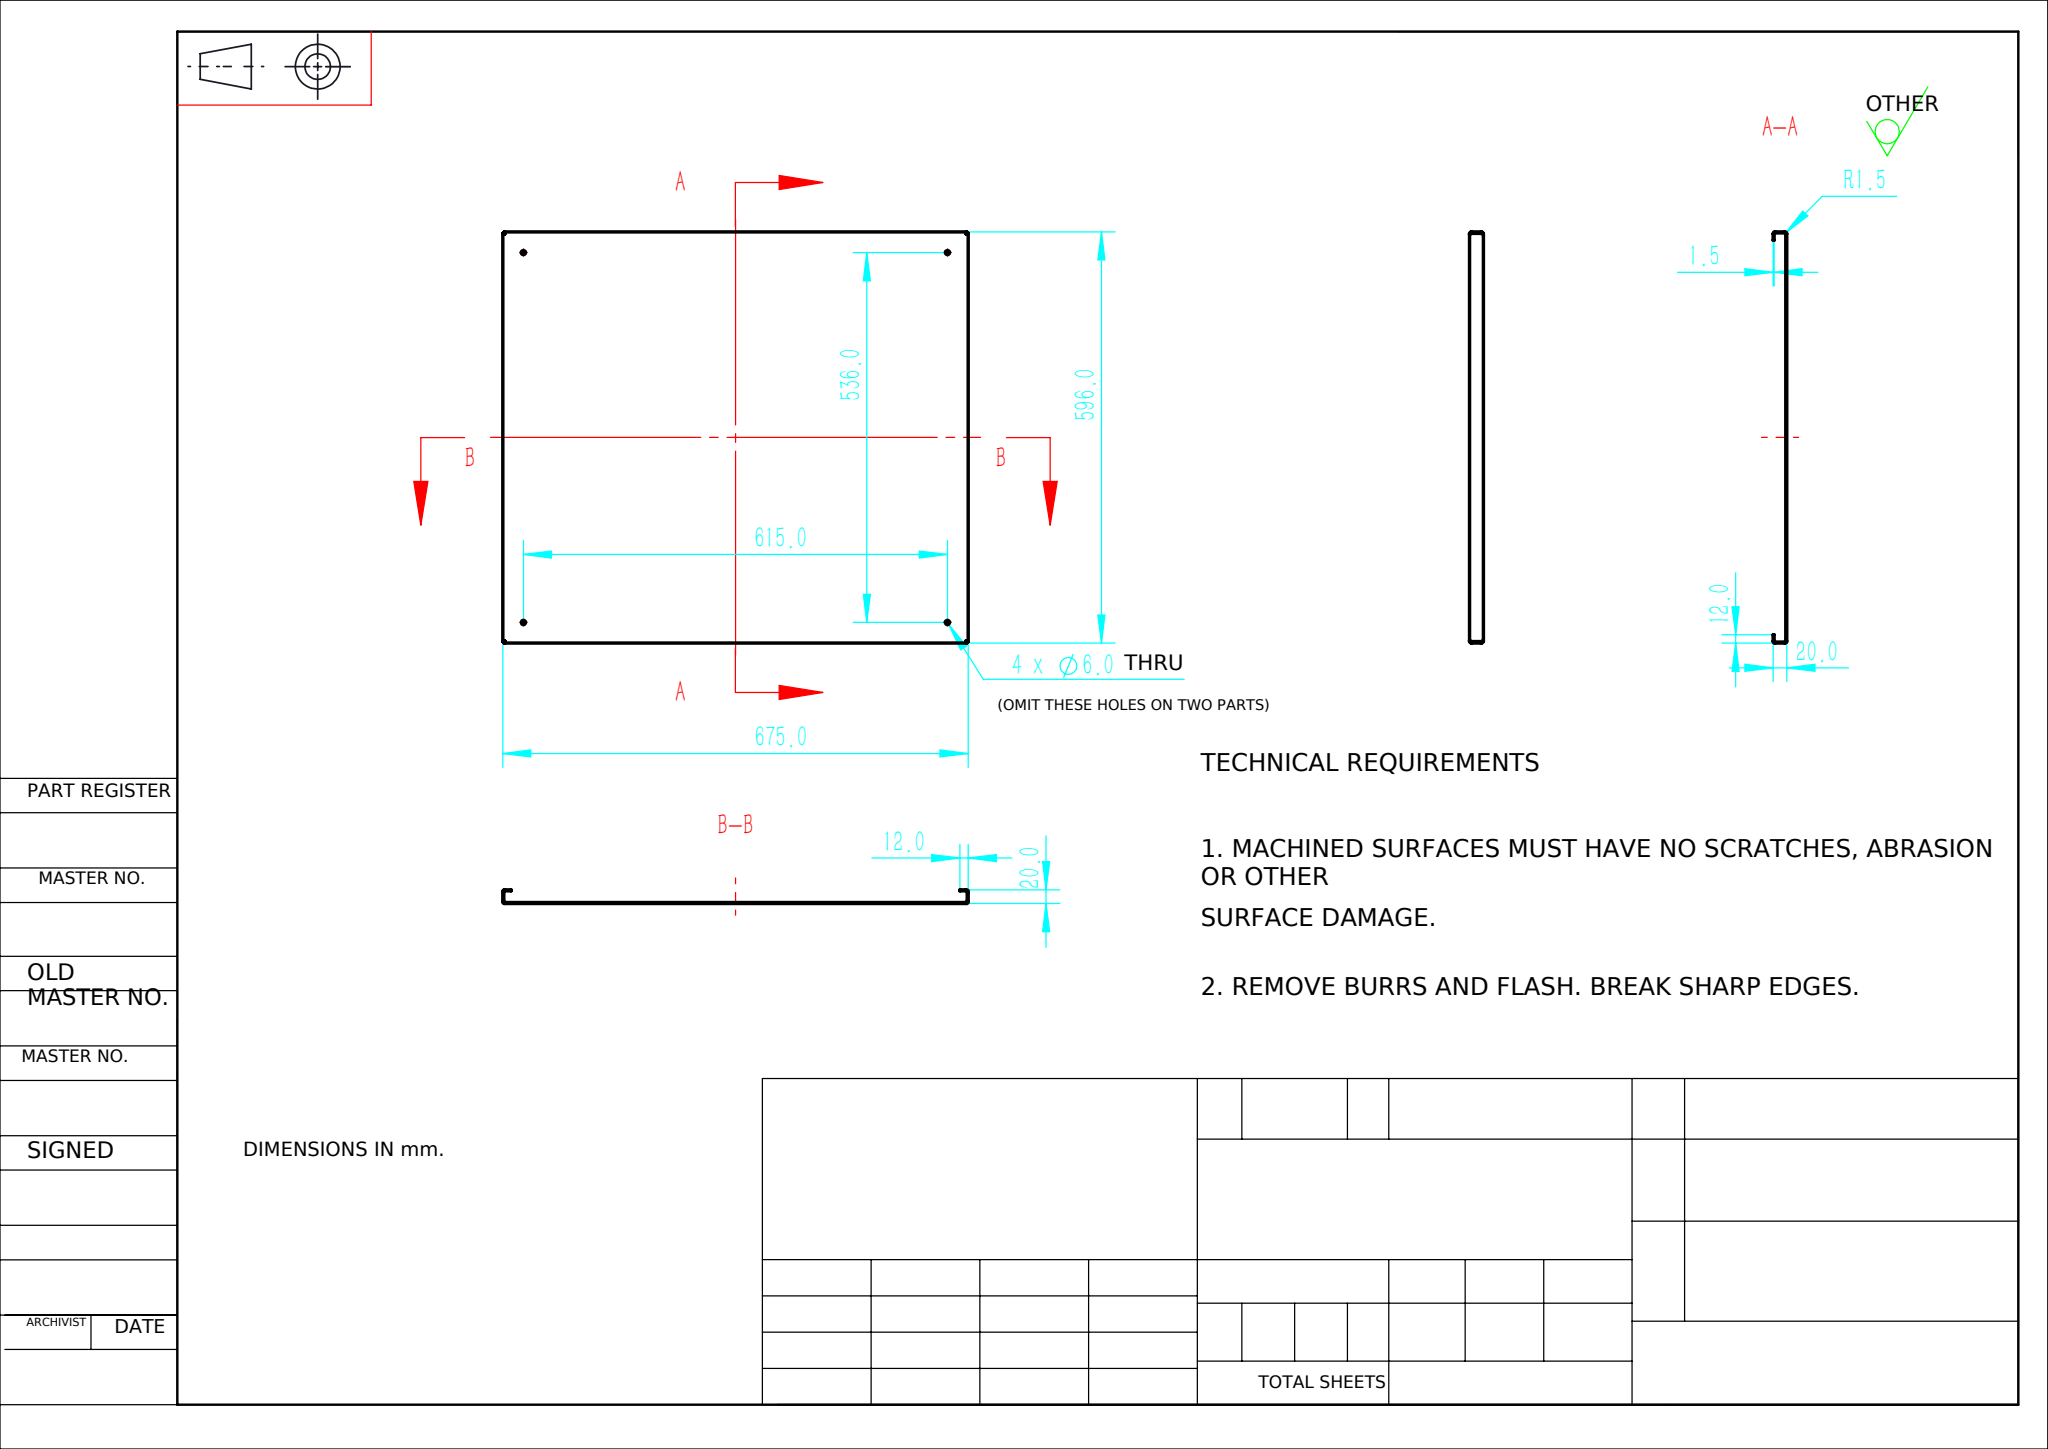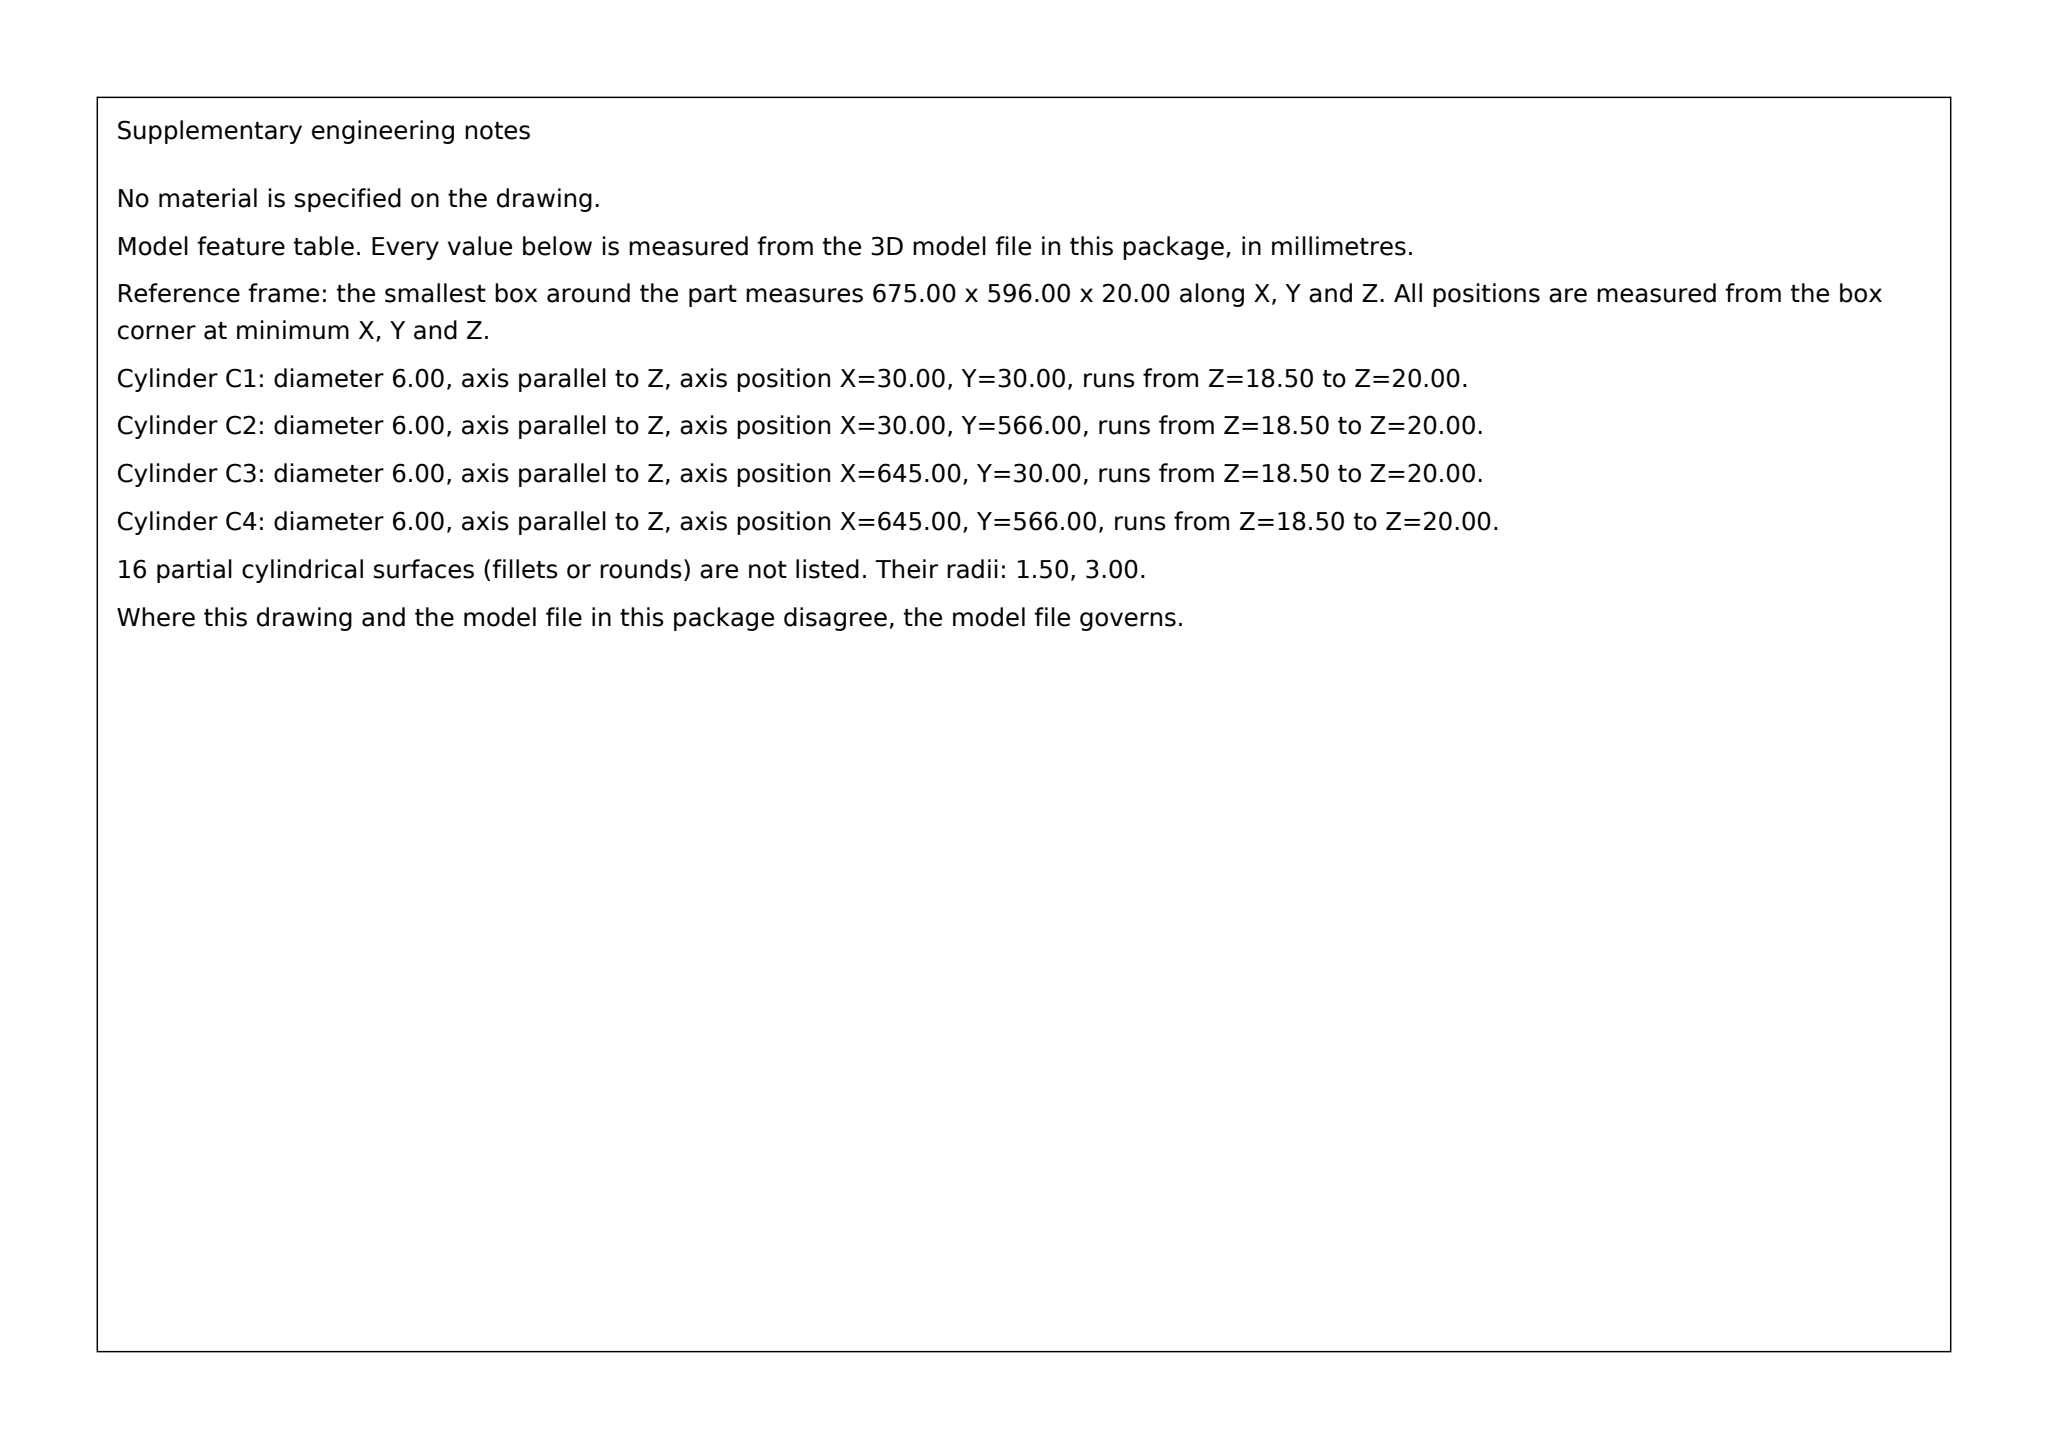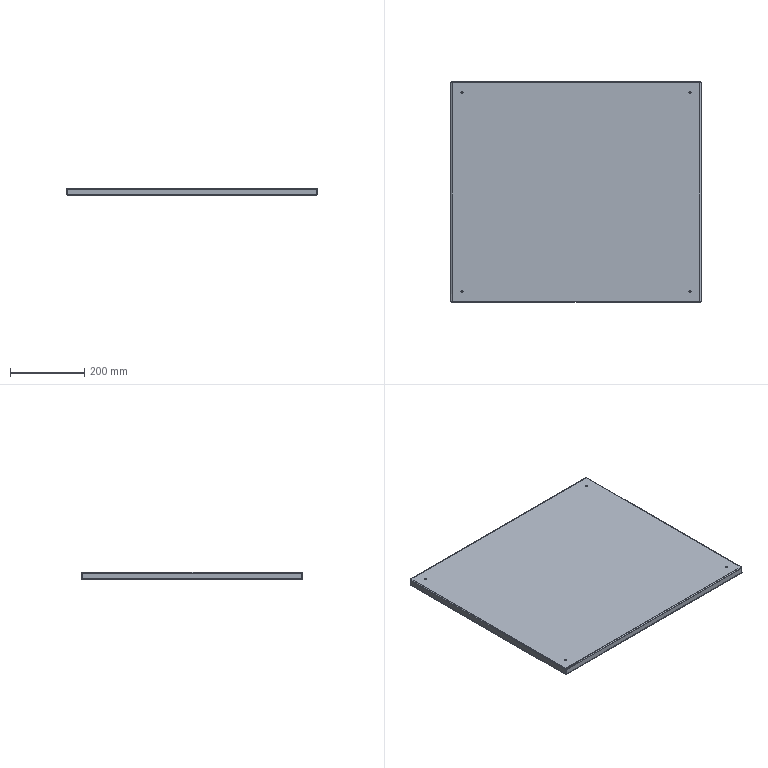Part | SolidWorks | mm | 1 solid | 78 faces | box 675 x 596 x 20 mm | volume 705054 mm3 | plane 38 | cylinder 24 | spline 16 | commonest cylinder face diameters 6 x16 3 x8